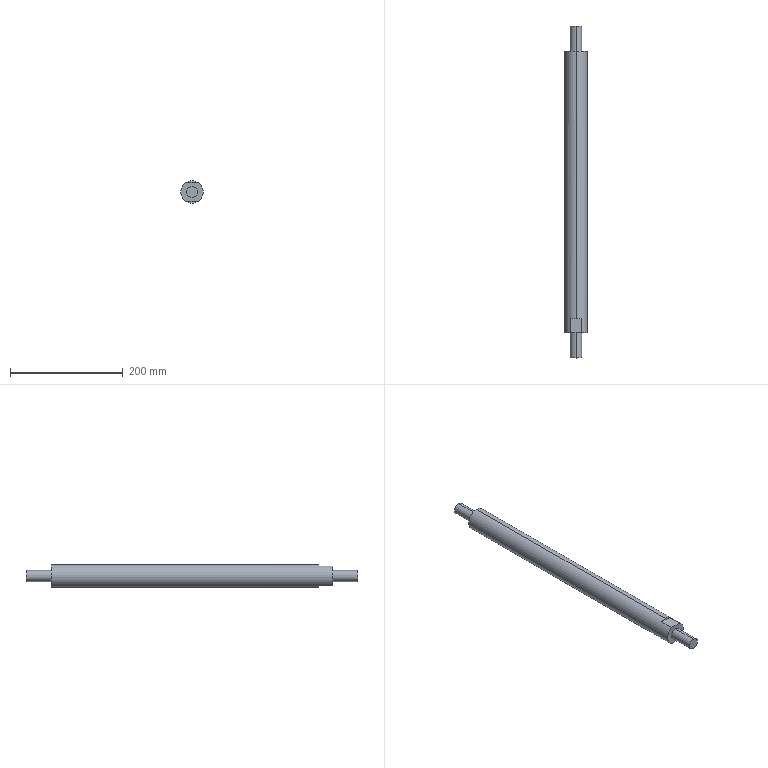Component | SolidWorks | -GuidePost-3 | 1 solid | 14 faces | box 40 x 590 x 40 mm | volume 654958 mm3 | plane 8 | cylinder 6 | commonest cylinder face diameters 20 x4 40 x2
build123d program:
from build123d import *

# Parameters (mm, degrees)
SKETCH2_W          = 10.42
SKETCH2_H          = 36.458
SKETCH2_W_2        = 14.312
SKETCH2_H_2        = 32.734
CUT_EXTRUDE1_DEPTH = 25


with BuildPart() as part:
    # Sketch1 → Revolve1 (revolve)
    with BuildSketch(Plane(origin=(0, 0, 0), x_dir=(1, 0, 0), z_dir=(0, 1, 0)), mode=Mode.PRIVATE) as revolve1_sk:
        Polygon((0, 0), (0, 10), (45, 10), (45, 20), (545, 20), (545, 10), (590, 10), (590, 0), align=None)
    revolve(revolve1_sk.sketch.rotate(Axis((-2616.332, 0, 0), (1, 0, 0)), 180), axis=Axis((-2616.332, 0, 0), (1, 0, 0)))

    # Sketch2 → Cut-Extrude1 (cut)
    with BuildSketch(Plane(origin=(545, 0, 0), x_dir=(0, 0, -1), z_dir=(1, 0, 0))):
        with Locations((-22.71, -0.09519)):
            Rectangle(SKETCH2_W, SKETCH2_H)
        with Locations((24.656, -1.298)):
            Rectangle(SKETCH2_W_2, SKETCH2_H_2)
    extrude(amount=-CUT_EXTRUDE1_DEPTH, mode=Mode.SUBTRACT)


solid = part.part

# Placed as in the assembly
solid = solid.moved(Location((-55, 1481, -40), (0, 0, -90)))
STEP:
#1=COLOUR_RGB('',0.7922,0.8196,0.9333);
#2=FILL_AREA_STYLE_COLOUR('',#1);
#3=FILL_AREA_STYLE('',(#2));
#4=SURFACE_STYLE_FILL_AREA(#3);
#5=SURFACE_SIDE_STYLE('',(#4));
#6=SURFACE_STYLE_USAGE(.BOTH.,#5);
#7=PRESENTATION_STYLE_ASSIGNMENT((#6));
#8=CARTESIAN_POINT('',(-2.165,35.079,-1.181));
#9=VERTEX_POINT('',#8);
#10=CARTESIAN_POINT('',(-2.165,35.079,-1.969));
#11=VERTEX_POINT('',#10);
#12=CARTESIAN_POINT('',(-2.165,35.079,-1.575));
#13=DIRECTION('',(0.,1.,-0.));
#14=DIRECTION('',(0.,0.,1.));
#15=AXIS2_PLACEMENT_3D('',#12,#13,#14);
#16=CIRCLE('',#15,0.3937);
#17=EDGE_CURVE('',#9,#11,#16,.T.);
#18=ORIENTED_EDGE('',*,*,#17,.T.);
#19=CARTESIAN_POINT('',(-2.165,36.85,-1.969));
#20=VERTEX_POINT('',#19);
#21=CARTESIAN_POINT('',(-2.165,161.312,-1.969));
#22=DIRECTION('',(0.,1.,-0.));
#23=VECTOR('',#22,39.37);
#24=LINE('',#21,#23);
#25=EDGE_CURVE('',#11,#20,#24,.T.);
#26=ORIENTED_EDGE('',*,*,#25,.T.);
#27=CARTESIAN_POINT('',(-2.165,36.85,-1.181));
#28=VERTEX_POINT('',#27);
#29=CARTESIAN_POINT('',(-2.165,36.85,-1.575));
#30=DIRECTION('',(0.,1.,-0.));
#31=DIRECTION('',(0.,0.,1.));
#32=AXIS2_PLACEMENT_3D('',#29,#30,#31);
#33=CIRCLE('',#32,0.3937);
#34=EDGE_CURVE('',#28,#20,#33,.T.);
#35=ORIENTED_EDGE('',*,*,#34,.F.);
#36=CARTESIAN_POINT('',(-2.165,161.312,-1.181));
#37=DIRECTION('',(0.,1.,-0.));
#38=VECTOR('',#37,39.37);
#39=LINE('',#36,#38);
#40=EDGE_CURVE('',#9,#28,#39,.T.);
#41=ORIENTED_EDGE('',*,*,#40,.F.);
#42=EDGE_LOOP('',(#18,#26,#35,#41));
#43=FACE_OUTER_BOUND('',#42,.T.);
#44=CARTESIAN_POINT('',(-2.165,161.312,-1.575));
#45=DIRECTION('',(0.,1.,-0.));
#46=DIRECTION('',(0.,0.,1.));
#47=AXIS2_PLACEMENT_3D('',#44,#45,#46);
#48=CYLINDRICAL_SURFACE('',#47,0.3937);
#49=ADVANCED_FACE('',(#43),#48,.T.);
#50=CARTESIAN_POINT('',(-1.784,37.835,-2.264));
#51=VERTEX_POINT('',#50);
#52=CARTESIAN_POINT('',(-2.165,37.835,-2.362));
#53=VERTEX_POINT('',#52);
#54=CARTESIAN_POINT('',(-2.165,37.835,-1.575));
#55=DIRECTION('',(0.,1.,-0.));
#56=DIRECTION('',(0.,0.,1.));
#57=AXIS2_PLACEMENT_3D('',#54,#55,#56);
#58=CIRCLE('',#57,0.7874);
#59=EDGE_CURVE('',#51,#53,#58,.T.);
#60=ORIENTED_EDGE('',*,*,#59,.T.);
#61=CARTESIAN_POINT('',(-2.165,56.535,-2.362));
#62=VERTEX_POINT('',#61);
#63=CARTESIAN_POINT('',(-2.165,161.312,-2.362));
#64=DIRECTION('',(0.,1.,-0.));
#65=VECTOR('',#64,39.37);
#66=LINE('',#63,#65);
#67=EDGE_CURVE('',#53,#62,#66,.T.);
#68=ORIENTED_EDGE('',*,*,#67,.T.);
#69=CARTESIAN_POINT('',(-2.165,56.535,-0.7874));
#70=VERTEX_POINT('',#69);
#71=CARTESIAN_POINT('',(-2.165,56.535,-1.575));
#72=DIRECTION('',(0.,1.,-0.));
#73=DIRECTION('',(0.,0.,1.));
#74=AXIS2_PLACEMENT_3D('',#71,#72,#73);
#75=CIRCLE('',#74,0.7874);
#76=EDGE_CURVE('',#70,#62,#75,.T.);
#77=ORIENTED_EDGE('',*,*,#76,.F.);
#78=CARTESIAN_POINT('',(-2.165,37.835,-0.7874));
#79=VERTEX_POINT('',#78);
#80=CARTESIAN_POINT('',(-2.165,161.312,-0.7874));
#81=DIRECTION('',(0.,1.,-0.));
#82=VECTOR('',#81,39.37);
#83=LINE('',#80,#82);
#84=EDGE_CURVE('',#79,#70,#83,.T.);
#85=ORIENTED_EDGE('',*,*,#84,.F.);
#86=CARTESIAN_POINT('',(-1.784,37.835,-0.8858));
#87=VERTEX_POINT('',#86);
#88=CARTESIAN_POINT('',(-2.165,37.835,-1.575));
#89=DIRECTION('',(-0.,-1.,0.));
#90=DIRECTION('',(0.,0.,-1.));
#91=AXIS2_PLACEMENT_3D('',#88,#89,#90);
#92=CIRCLE('',#91,0.7874);
#93=EDGE_CURVE('',#87,#79,#92,.T.);
#94=ORIENTED_EDGE('',*,*,#93,.F.);
#95=CARTESIAN_POINT('',(-1.784,36.85,-0.8858));
#96=VERTEX_POINT('',#95);
#97=CARTESIAN_POINT('',(-1.784,161.312,-0.8858));
#98=DIRECTION('',(-0.,-1.,0.));
#99=VECTOR('',#98,39.37);
#100=LINE('',#97,#99);
#101=EDGE_CURVE('',#87,#96,#100,.T.);
#102=ORIENTED_EDGE('',*,*,#101,.T.);
#103=CARTESIAN_POINT('',(-1.784,36.85,-2.264));
#104=VERTEX_POINT('',#103);
#105=CARTESIAN_POINT('',(-2.165,36.85,-1.575));
#106=DIRECTION('',(0.,1.,-0.));
#107=DIRECTION('',(0.,0.,1.));
#108=AXIS2_PLACEMENT_3D('',#105,#106,#107);
#109=CIRCLE('',#108,0.7874);
#110=EDGE_CURVE('',#96,#104,#109,.T.);
#111=ORIENTED_EDGE('',*,*,#110,.T.);
#112=CARTESIAN_POINT('',(-1.784,161.312,-2.264));
#113=DIRECTION('',(0.,1.,-0.));
#114=VECTOR('',#113,39.37);
#115=LINE('',#112,#114);
#116=EDGE_CURVE('',#104,#51,#115,.T.);
#117=ORIENTED_EDGE('',*,*,#116,.T.);
#118=EDGE_LOOP('',(#60,#68,#77,#85,#94,#102,#111,#117));
#119=FACE_OUTER_BOUND('',#118,.T.);
#120=CARTESIAN_POINT('',(-2.165,161.312,-1.575));
#121=DIRECTION('',(0.,1.,-0.));
#122=DIRECTION('',(0.,0.,1.));
#123=AXIS2_PLACEMENT_3D('',#120,#121,#122);
#124=CYLINDRICAL_SURFACE('',#123,0.7874);
#125=ADVANCED_FACE('',(#119),#124,.T.);
#126=CARTESIAN_POINT('',(-2.165,56.535,-1.181));
#127=VERTEX_POINT('',#126);
#128=CARTESIAN_POINT('',(-2.165,56.535,-1.969));
#129=VERTEX_POINT('',#128);
#130=CARTESIAN_POINT('',(-2.165,56.535,-1.575));
#131=DIRECTION('',(0.,1.,-0.));
#132=DIRECTION('',(0.,0.,1.));
#133=AXIS2_PLACEMENT_3D('',#130,#131,#132);
#134=CIRCLE('',#133,0.3937);
#135=EDGE_CURVE('',#127,#129,#134,.T.);
#136=ORIENTED_EDGE('',*,*,#135,.T.);
#137=CARTESIAN_POINT('',(-2.165,58.307,-1.969));
#138=VERTEX_POINT('',#137);
#139=CARTESIAN_POINT('',(-2.165,161.312,-1.969));
#140=DIRECTION('',(0.,1.,-0.));
#141=VECTOR('',#140,39.37);
#142=LINE('',#139,#141);
#143=EDGE_CURVE('',#129,#138,#142,.T.);
#144=ORIENTED_EDGE('',*,*,#143,.T.);
#145=CARTESIAN_POINT('',(-2.165,58.307,-1.181));
#146=VERTEX_POINT('',#145);
#147=CARTESIAN_POINT('',(-2.165,58.307,-1.575));
#148=DIRECTION('',(0.,1.,-0.));
#149=DIRECTION('',(0.,0.,1.));
#150=AXIS2_PLACEMENT_3D('',#147,#148,#149);
#151=CIRCLE('',#150,0.3937);
#152=EDGE_CURVE('',#146,#138,#151,.T.);
#153=ORIENTED_EDGE('',*,*,#152,.F.);
#154=CARTESIAN_POINT('',(-2.165,161.312,-1.181));
#155=DIRECTION('',(0.,1.,-0.));
#156=VECTOR('',#155,39.37);
#157=LINE('',#154,#156);
#158=EDGE_CURVE('',#127,#146,#157,.T.);
#159=ORIENTED_EDGE('',*,*,#158,.F.);
#160=EDGE_LOOP('',(#136,#144,#153,#159));
#161=FACE_OUTER_BOUND('',#160,.T.);
#162=CARTESIAN_POINT('',(-2.165,161.312,-1.575));
#163=DIRECTION('',(0.,1.,-0.));
#164=DIRECTION('',(0.,0.,1.));
#165=AXIS2_PLACEMENT_3D('',#162,#163,#164);
#166=CYLINDRICAL_SURFACE('',#165,0.3937);
#167=ADVANCED_FACE('',(#161),#166,.T.);
#168=ORIENTED_EDGE('',*,*,#152,.T.);
#169=CARTESIAN_POINT('',(-2.165,58.307,-1.575));
#170=DIRECTION('',(0.,1.,-0.));
#171=DIRECTION('',(0.,0.,1.));
#172=AXIS2_PLACEMENT_3D('',#169,#170,#171);
#173=CIRCLE('',#172,0.3937);
#174=EDGE_CURVE('',#138,#146,#173,.T.);
#175=ORIENTED_EDGE('',*,*,#174,.T.);
#176=EDGE_LOOP('',(#168,#175));
#177=FACE_OUTER_BOUND('',#176,.T.);
#178=CARTESIAN_POINT('',(-2.165,58.307,-1.575));
#179=DIRECTION('',(-0.,-1.,0.));
#180=DIRECTION('',(0.,-0.,-1.));
#181=AXIS2_PLACEMENT_3D('',#178,#179,#180);
#182=PLANE('',#181);
#183=ADVANCED_FACE('',(#177),#182,.F.);
#184=ORIENTED_EDGE('',*,*,#143,.F.);
#185=CARTESIAN_POINT('',(-2.165,56.535,-1.575));
#186=DIRECTION('',(0.,1.,-0.));
#187=DIRECTION('',(0.,0.,1.));
#188=AXIS2_PLACEMENT_3D('',#185,#186,#187);
#189=CIRCLE('',#188,0.3937);
#190=EDGE_CURVE('',#129,#127,#189,.T.);
#191=ORIENTED_EDGE('',*,*,#190,.T.);
#192=ORIENTED_EDGE('',*,*,#158,.T.);
#193=ORIENTED_EDGE('',*,*,#174,.F.);
#194=EDGE_LOOP('',(#184,#191,#192,#193));
#195=FACE_OUTER_BOUND('',#194,.T.);
#196=CARTESIAN_POINT('',(-2.165,161.312,-1.575));
#197=DIRECTION('',(0.,1.,-0.));
#198=DIRECTION('',(0.,0.,1.));
#199=AXIS2_PLACEMENT_3D('',#196,#197,#198);
#200=CYLINDRICAL_SURFACE('',#199,0.3937);
#201=ADVANCED_FACE('',(#195),#200,.T.);
#202=ORIENTED_EDGE('',*,*,#135,.F.);
#203=ORIENTED_EDGE('',*,*,#190,.F.);
#204=EDGE_LOOP('',(#202,#203));
#205=FACE_BOUND('',#204,.T.);
#206=ORIENTED_EDGE('',*,*,#76,.T.);
#207=CARTESIAN_POINT('',(-2.165,56.535,-1.575));
#208=DIRECTION('',(0.,1.,-0.));
#209=DIRECTION('',(0.,0.,1.));
#210=AXIS2_PLACEMENT_3D('',#207,#208,#209);
#211=CIRCLE('',#210,0.7874);
#212=EDGE_CURVE('',#62,#70,#211,.T.);
#213=ORIENTED_EDGE('',*,*,#212,.T.);
#214=EDGE_LOOP('',(#206,#213));
#215=FACE_OUTER_BOUND('',#214,.T.);
#216=CARTESIAN_POINT('',(-2.165,56.535,-1.969));
#217=DIRECTION('',(-0.,-1.,0.));
#218=DIRECTION('',(0.,-0.,-1.));
#219=AXIS2_PLACEMENT_3D('',#216,#217,#218);
#220=PLANE('',#219);
#221=ADVANCED_FACE('',(#205,#215),#220,.F.);
#222=ORIENTED_EDGE('',*,*,#67,.F.);
#223=CARTESIAN_POINT('',(-2.547,37.835,-2.264));
#224=VERTEX_POINT('',#223);
#225=CARTESIAN_POINT('',(-2.165,37.835,-1.575));
#226=DIRECTION('',(0.,1.,-0.));
#227=DIRECTION('',(0.,0.,1.));
#228=AXIS2_PLACEMENT_3D('',#225,#226,#227);
#229=CIRCLE('',#228,0.7874);
#230=EDGE_CURVE('',#53,#224,#229,.T.);
#231=ORIENTED_EDGE('',*,*,#230,.T.);
#232=CARTESIAN_POINT('',(-2.547,36.85,-2.264));
#233=VERTEX_POINT('',#232);
#234=CARTESIAN_POINT('',(-2.547,161.312,-2.264));
#235=DIRECTION('',(-0.,-1.,0.));
#236=VECTOR('',#235,39.37);
#237=LINE('',#234,#236);
#238=EDGE_CURVE('',#224,#233,#237,.T.);
#239=ORIENTED_EDGE('',*,*,#238,.T.);
#240=CARTESIAN_POINT('',(-2.547,36.85,-0.8858));
#241=VERTEX_POINT('',#240);
#242=CARTESIAN_POINT('',(-2.165,36.85,-1.575));
#243=DIRECTION('',(0.,1.,-0.));
#244=DIRECTION('',(0.,0.,1.));
#245=AXIS2_PLACEMENT_3D('',#242,#243,#244);
#246=CIRCLE('',#245,0.7874);
#247=EDGE_CURVE('',#233,#241,#246,.T.);
#248=ORIENTED_EDGE('',*,*,#247,.T.);
#249=CARTESIAN_POINT('',(-2.547,37.835,-0.8858));
#250=VERTEX_POINT('',#249);
#251=CARTESIAN_POINT('',(-2.547,161.312,-0.8858));
#252=DIRECTION('',(0.,1.,-0.));
#253=VECTOR('',#252,39.37);
#254=LINE('',#251,#253);
#255=EDGE_CURVE('',#241,#250,#254,.T.);
#256=ORIENTED_EDGE('',*,*,#255,.T.);
#257=CARTESIAN_POINT('',(-2.165,37.835,-1.575));
#258=DIRECTION('',(-0.,-1.,0.));
#259=DIRECTION('',(0.,0.,-1.));
#260=AXIS2_PLACEMENT_3D('',#257,#258,#259);
#261=CIRCLE('',#260,0.7874);
#262=EDGE_CURVE('',#79,#250,#261,.T.);
#263=ORIENTED_EDGE('',*,*,#262,.F.);
#264=ORIENTED_EDGE('',*,*,#84,.T.);
#265=ORIENTED_EDGE('',*,*,#212,.F.);
#266=EDGE_LOOP('',(#222,#231,#239,#248,#256,#263,#264,#265));
#267=FACE_OUTER_BOUND('',#266,.T.);
#268=CARTESIAN_POINT('',(-2.165,161.312,-1.575));
#269=DIRECTION('',(0.,1.,-0.));
#270=DIRECTION('',(0.,0.,1.));
#271=AXIS2_PLACEMENT_3D('',#268,#269,#270);
#272=CYLINDRICAL_SURFACE('',#271,0.7874);
#273=ADVANCED_FACE('',(#267),#272,.T.);
#274=ORIENTED_EDGE('',*,*,#247,.F.);
#275=CARTESIAN_POINT('',(-2.165,36.85,-2.264));
#276=DIRECTION('',(1.,0.,0.));
#277=VECTOR('',#276,39.37);
#278=LINE('',#275,#277);
#279=EDGE_CURVE('',#233,#104,#278,.T.);
#280=ORIENTED_EDGE('',*,*,#279,.T.);
#281=ORIENTED_EDGE('',*,*,#110,.F.);
#282=CARTESIAN_POINT('',(-2.165,36.85,-0.8858));
#283=DIRECTION('',(-1.,-0.,-0.));
#284=VECTOR('',#283,39.37);
#285=LINE('',#282,#284);
#286=EDGE_CURVE('',#96,#241,#285,.T.);
#287=ORIENTED_EDGE('',*,*,#286,.T.);
#288=EDGE_LOOP('',(#274,#280,#281,#287));
#289=FACE_OUTER_BOUND('',#288,.T.);
#290=ORIENTED_EDGE('',*,*,#34,.T.);
#291=CARTESIAN_POINT('',(-2.165,36.85,-1.575));
#292=DIRECTION('',(0.,1.,-0.));
#293=DIRECTION('',(0.,0.,1.));
#294=AXIS2_PLACEMENT_3D('',#291,#292,#293);
#295=CIRCLE('',#294,0.3937);
#296=EDGE_CURVE('',#20,#28,#295,.T.);
#297=ORIENTED_EDGE('',*,*,#296,.T.);
#298=EDGE_LOOP('',(#290,#297));
#299=FACE_BOUND('',#298,.T.);
#300=CARTESIAN_POINT('',(-2.165,36.85,-2.362));
#301=DIRECTION('',(0.,1.,-0.));
#302=DIRECTION('',(0.,0.,1.));
#303=AXIS2_PLACEMENT_3D('',#300,#301,#302);
#304=PLANE('',#303);
#305=ADVANCED_FACE('',(#289,#299),#304,.F.);
#306=ORIENTED_EDGE('',*,*,#25,.F.);
#307=CARTESIAN_POINT('',(-2.165,35.079,-1.575));
#308=DIRECTION('',(0.,1.,-0.));
#309=DIRECTION('',(0.,0.,1.));
#310=AXIS2_PLACEMENT_3D('',#307,#308,#309);
#311=CIRCLE('',#310,0.3937);
#312=EDGE_CURVE('',#11,#9,#311,.T.);
#313=ORIENTED_EDGE('',*,*,#312,.T.);
#314=ORIENTED_EDGE('',*,*,#40,.T.);
#315=ORIENTED_EDGE('',*,*,#296,.F.);
#316=EDGE_LOOP('',(#306,#313,#314,#315));
#317=FACE_OUTER_BOUND('',#316,.T.);
#318=CARTESIAN_POINT('',(-2.165,161.312,-1.575));
#319=DIRECTION('',(0.,1.,-0.));
#320=DIRECTION('',(0.,0.,1.));
#321=AXIS2_PLACEMENT_3D('',#318,#319,#320);
#322=CYLINDRICAL_SURFACE('',#321,0.3937);
#323=ADVANCED_FACE('',(#317),#322,.T.);
#324=ORIENTED_EDGE('',*,*,#17,.F.);
#325=ORIENTED_EDGE('',*,*,#312,.F.);
#326=EDGE_LOOP('',(#324,#325));
#327=FACE_OUTER_BOUND('',#326,.T.);
#328=CARTESIAN_POINT('',(-2.165,35.079,-1.969));
#329=DIRECTION('',(0.,1.,-0.));
#330=DIRECTION('',(0.,0.,1.));
#331=AXIS2_PLACEMENT_3D('',#328,#329,#330);
#332=PLANE('',#331);
#333=ADVANCED_FACE('',(#327),#332,.F.);
#334=ORIENTED_EDGE('',*,*,#93,.T.);
#335=ORIENTED_EDGE('',*,*,#262,.T.);
#336=CARTESIAN_POINT('',(-1.451,37.835,-0.8858));
#337=DIRECTION('',(1.,0.,0.));
#338=VECTOR('',#337,39.37);
#339=LINE('',#336,#338);
#340=EDGE_CURVE('',#250,#87,#339,.T.);
#341=ORIENTED_EDGE('',*,*,#340,.T.);
#342=EDGE_LOOP('',(#334,#335,#341));
#343=FACE_OUTER_BOUND('',#342,.T.);
#344=CARTESIAN_POINT('',(-2.165,37.835,-1.575));
#345=DIRECTION('',(-0.,-1.,0.));
#346=DIRECTION('',(0.,-0.,-1.));
#347=AXIS2_PLACEMENT_3D('',#344,#345,#346);
#348=PLANE('',#347);
#349=ADVANCED_FACE('',(#343),#348,.T.);
#350=ORIENTED_EDGE('',*,*,#286,.F.);
#351=ORIENTED_EDGE('',*,*,#101,.F.);
#352=ORIENTED_EDGE('',*,*,#340,.F.);
#353=ORIENTED_EDGE('',*,*,#255,.F.);
#354=EDGE_LOOP('',(#350,#351,#352,#353));
#355=FACE_OUTER_BOUND('',#354,.T.);
#356=CARTESIAN_POINT('',(-1.451,37.835,-0.8858));
#357=DIRECTION('',(0.,-0.,-1.));
#358=DIRECTION('',(1.,0.,0.));
#359=AXIS2_PLACEMENT_3D('',#356,#357,#358);
#360=PLANE('',#359);
#361=ADVANCED_FACE('',(#355),#360,.F.);
#362=CARTESIAN_POINT('',(-1.572,37.835,-2.264));
#363=DIRECTION('',(-1.,-0.,-0.));
#364=VECTOR('',#363,39.37);
#365=LINE('',#362,#364);
#366=EDGE_CURVE('',#51,#224,#365,.T.);
#367=ORIENTED_EDGE('',*,*,#366,.T.);
#368=ORIENTED_EDGE('',*,*,#230,.F.);
#369=ORIENTED_EDGE('',*,*,#59,.F.);
#370=EDGE_LOOP('',(#367,#368,#369));
#371=FACE_OUTER_BOUND('',#370,.T.);
#372=CARTESIAN_POINT('',(-2.165,37.835,-1.575));
#373=DIRECTION('',(0.,1.,-0.));
#374=DIRECTION('',(0.,0.,1.));
#375=AXIS2_PLACEMENT_3D('',#372,#373,#374);
#376=PLANE('',#375);
#377=ADVANCED_FACE('',(#371),#376,.F.);
#378=ORIENTED_EDGE('',*,*,#279,.F.);
#379=ORIENTED_EDGE('',*,*,#238,.F.);
#380=ORIENTED_EDGE('',*,*,#366,.F.);
#381=ORIENTED_EDGE('',*,*,#116,.F.);
#382=EDGE_LOOP('',(#378,#379,#380,#381));
#383=FACE_OUTER_BOUND('',#382,.T.);
#384=CARTESIAN_POINT('',(-1.572,37.835,-2.264));
#385=DIRECTION('',(-0.,0.,1.));
#386=DIRECTION('',(-1.,-0.,-0.));
#387=AXIS2_PLACEMENT_3D('',#384,#385,#386);
#388=PLANE('',#387);
#389=ADVANCED_FACE('',(#383),#388,.F.);
#390=CLOSED_SHELL('',(#49,#125,#167,#183,#201,#221,#273,#305,#323,#333,#349,#361,#377,#389));
#391=MANIFOLD_SOLID_BREP('',#390);
#392=STYLED_ITEM('',(#7),#391);
#393=PRESENTATION_LAYER_ASSIGNMENT('','',(#392));
#394=(LENGTH_UNIT()NAMED_UNIT(*)SI_UNIT($,.METRE.));
#395=LENGTH_MEASURE_WITH_UNIT(LENGTH_MEASURE(0.0254),#394);
#396=DIMENSIONAL_EXPONENTS(1.,0.,0.,0.,0.,0.,0.);
#397=(CONVERSION_BASED_UNIT('',#395)LENGTH_UNIT()NAMED_UNIT(#396));
#398=UNCERTAINTY_MEASURE_WITH_UNIT(LENGTH_MEASURE(0.00001),#397,'','');
#399=(NAMED_UNIT(*)PLANE_ANGLE_UNIT()SI_UNIT($,.RADIAN.));
#400=(NAMED_UNIT(*)SI_UNIT($,.STERADIAN.)SOLID_ANGLE_UNIT());
#401=(GEOMETRIC_REPRESENTATION_CONTEXT(3)GLOBAL_UNCERTAINTY_ASSIGNED_CONTEXT((#398))GLOBAL_UNIT_ASSIGNED_CONTEXT((#397,#399,#400))REPRESENTATION_CONTEXT('',''));
#402=MECHANICAL_DESIGN_GEOMETRIC_PRESENTATION_REPRESENTATION('',(#392),#401);
#403=CARTESIAN_POINT('',(0.,0.,0.));
#404=DIRECTION('',(0.,0.,1.));
#405=DIRECTION('',(1.,0.,0.));
#406=AXIS2_PLACEMENT_3D('',#403,#404,#405);
#407=(LENGTH_UNIT()NAMED_UNIT(*)SI_UNIT($,.METRE.));
#408=LENGTH_MEASURE_WITH_UNIT(LENGTH_MEASURE(0.0254),#407);
#409=DIMENSIONAL_EXPONENTS(1.,0.,0.,0.,0.,0.,0.);
#410=(CONVERSION_BASED_UNIT('',#408)LENGTH_UNIT()NAMED_UNIT(#409));
#411=UNCERTAINTY_MEASURE_WITH_UNIT(LENGTH_MEASURE(0.00001),#410,'','');
#412=(NAMED_UNIT(*)PLANE_ANGLE_UNIT()SI_UNIT($,.RADIAN.));
#413=(NAMED_UNIT(*)SI_UNIT($,.STERADIAN.)SOLID_ANGLE_UNIT());
#414=(GEOMETRIC_REPRESENTATION_CONTEXT(3)GLOBAL_UNCERTAINTY_ASSIGNED_CONTEXT((#411))GLOBAL_UNIT_ASSIGNED_CONTEXT((#410,#412,#413))REPRESENTATION_CONTEXT('',''));
#415=ADVANCED_BREP_SHAPE_REPRESENTATION('',(#391,#406),#414);